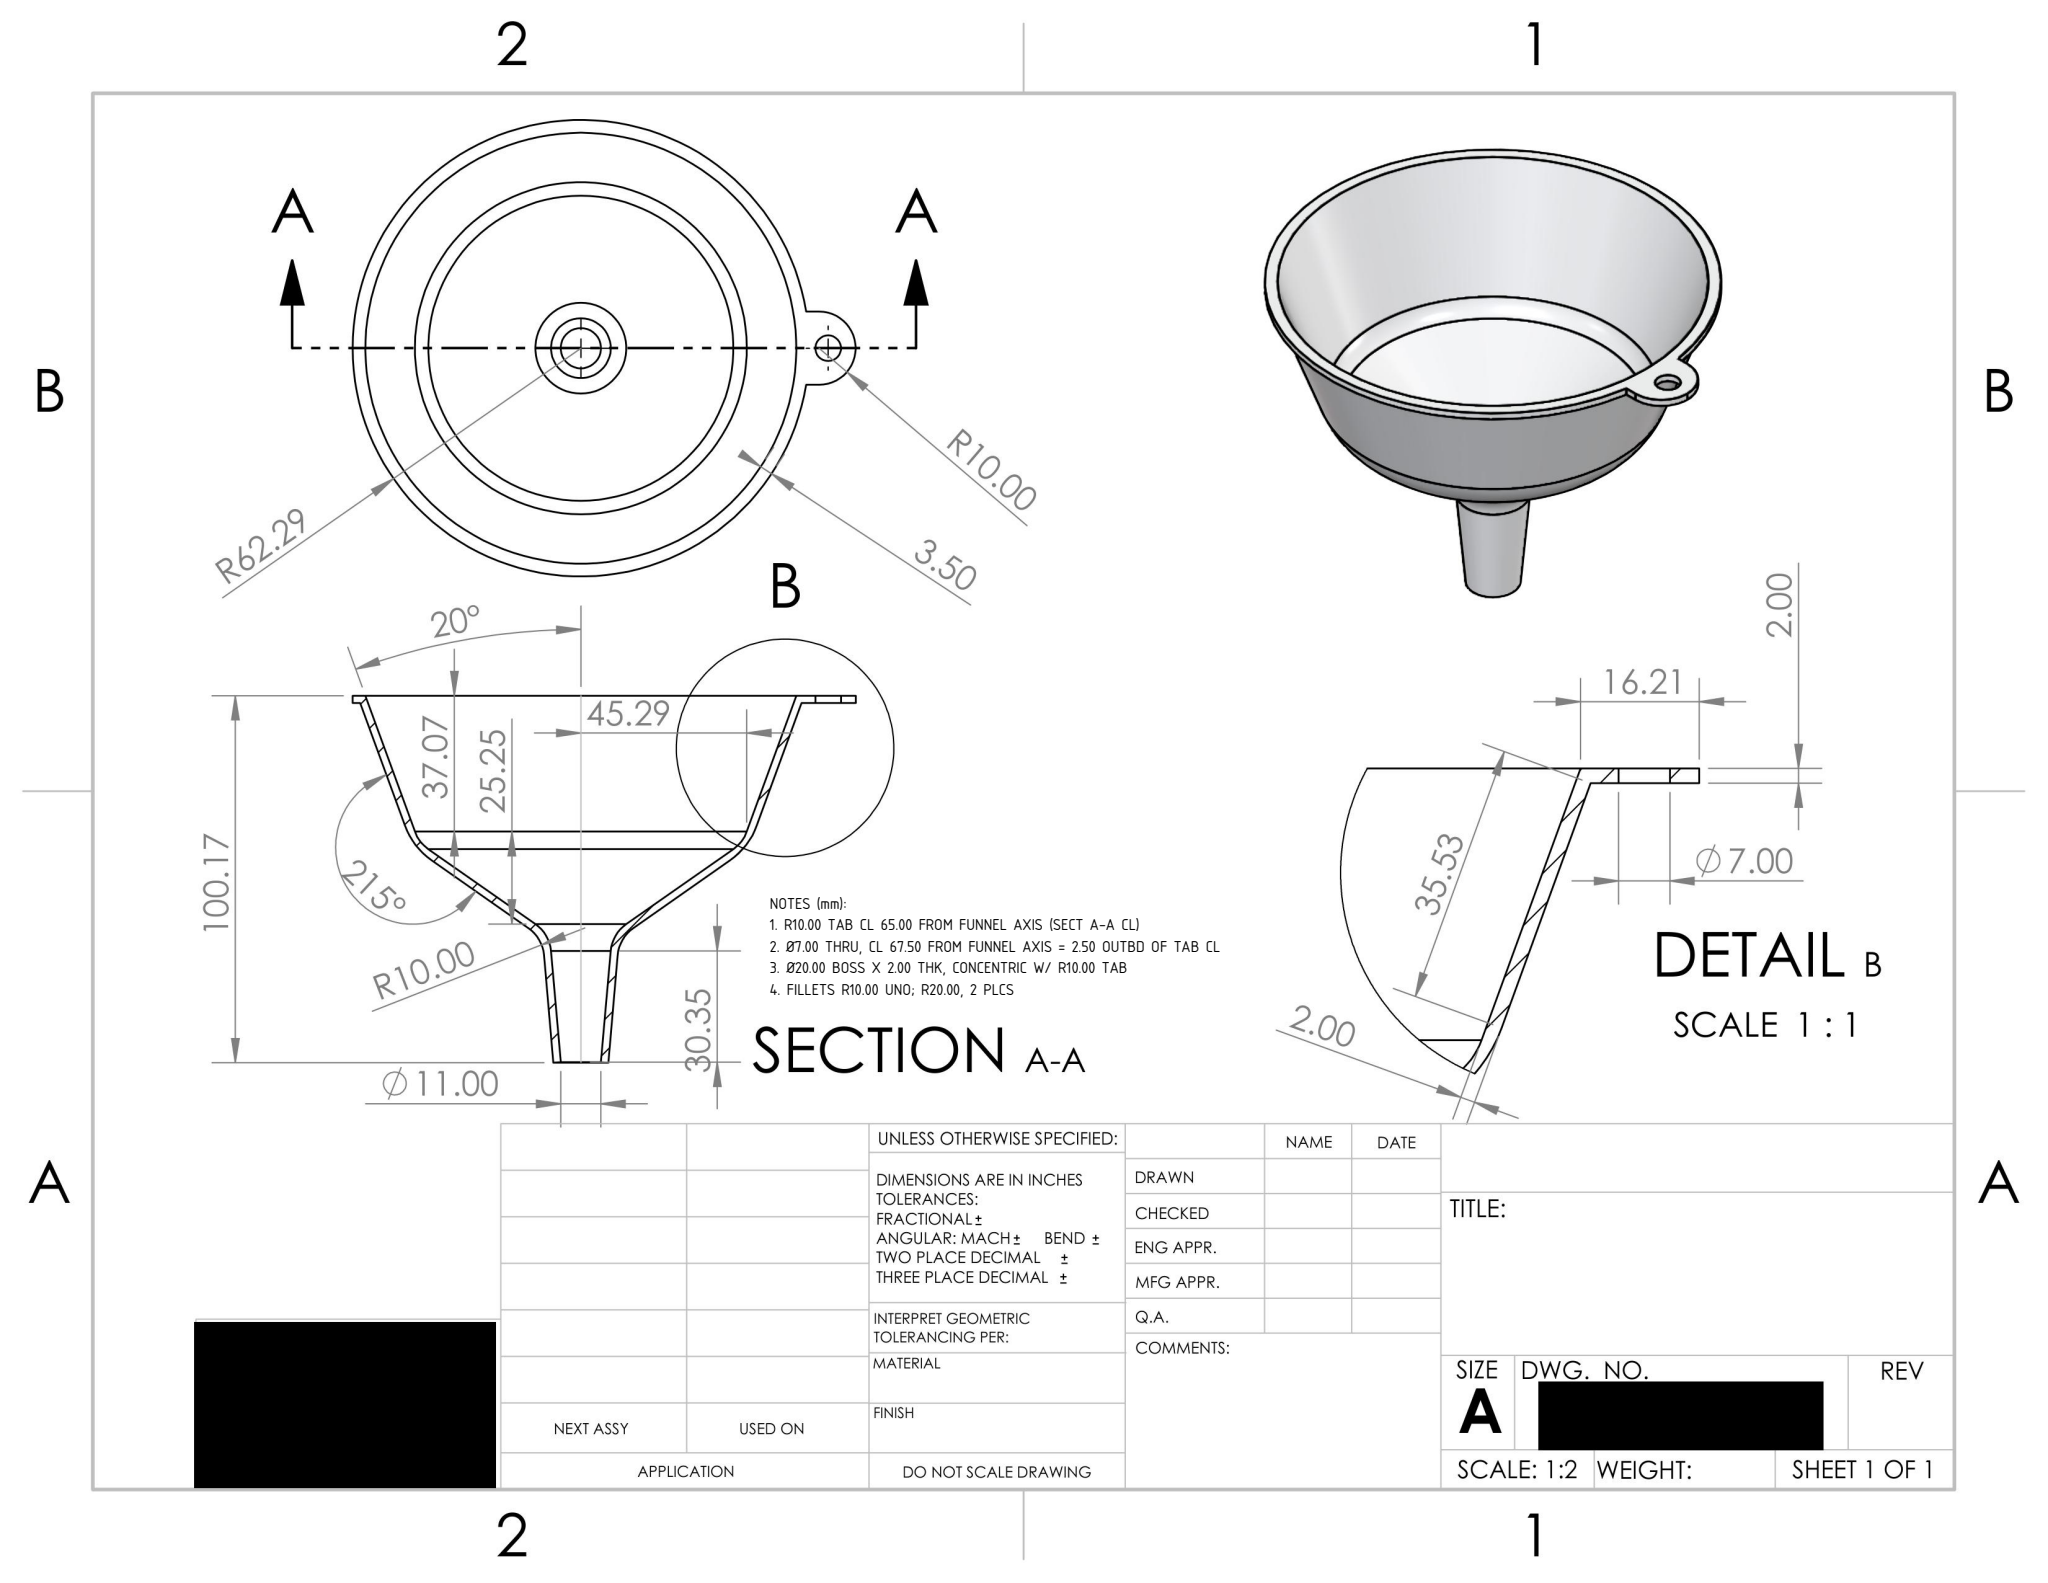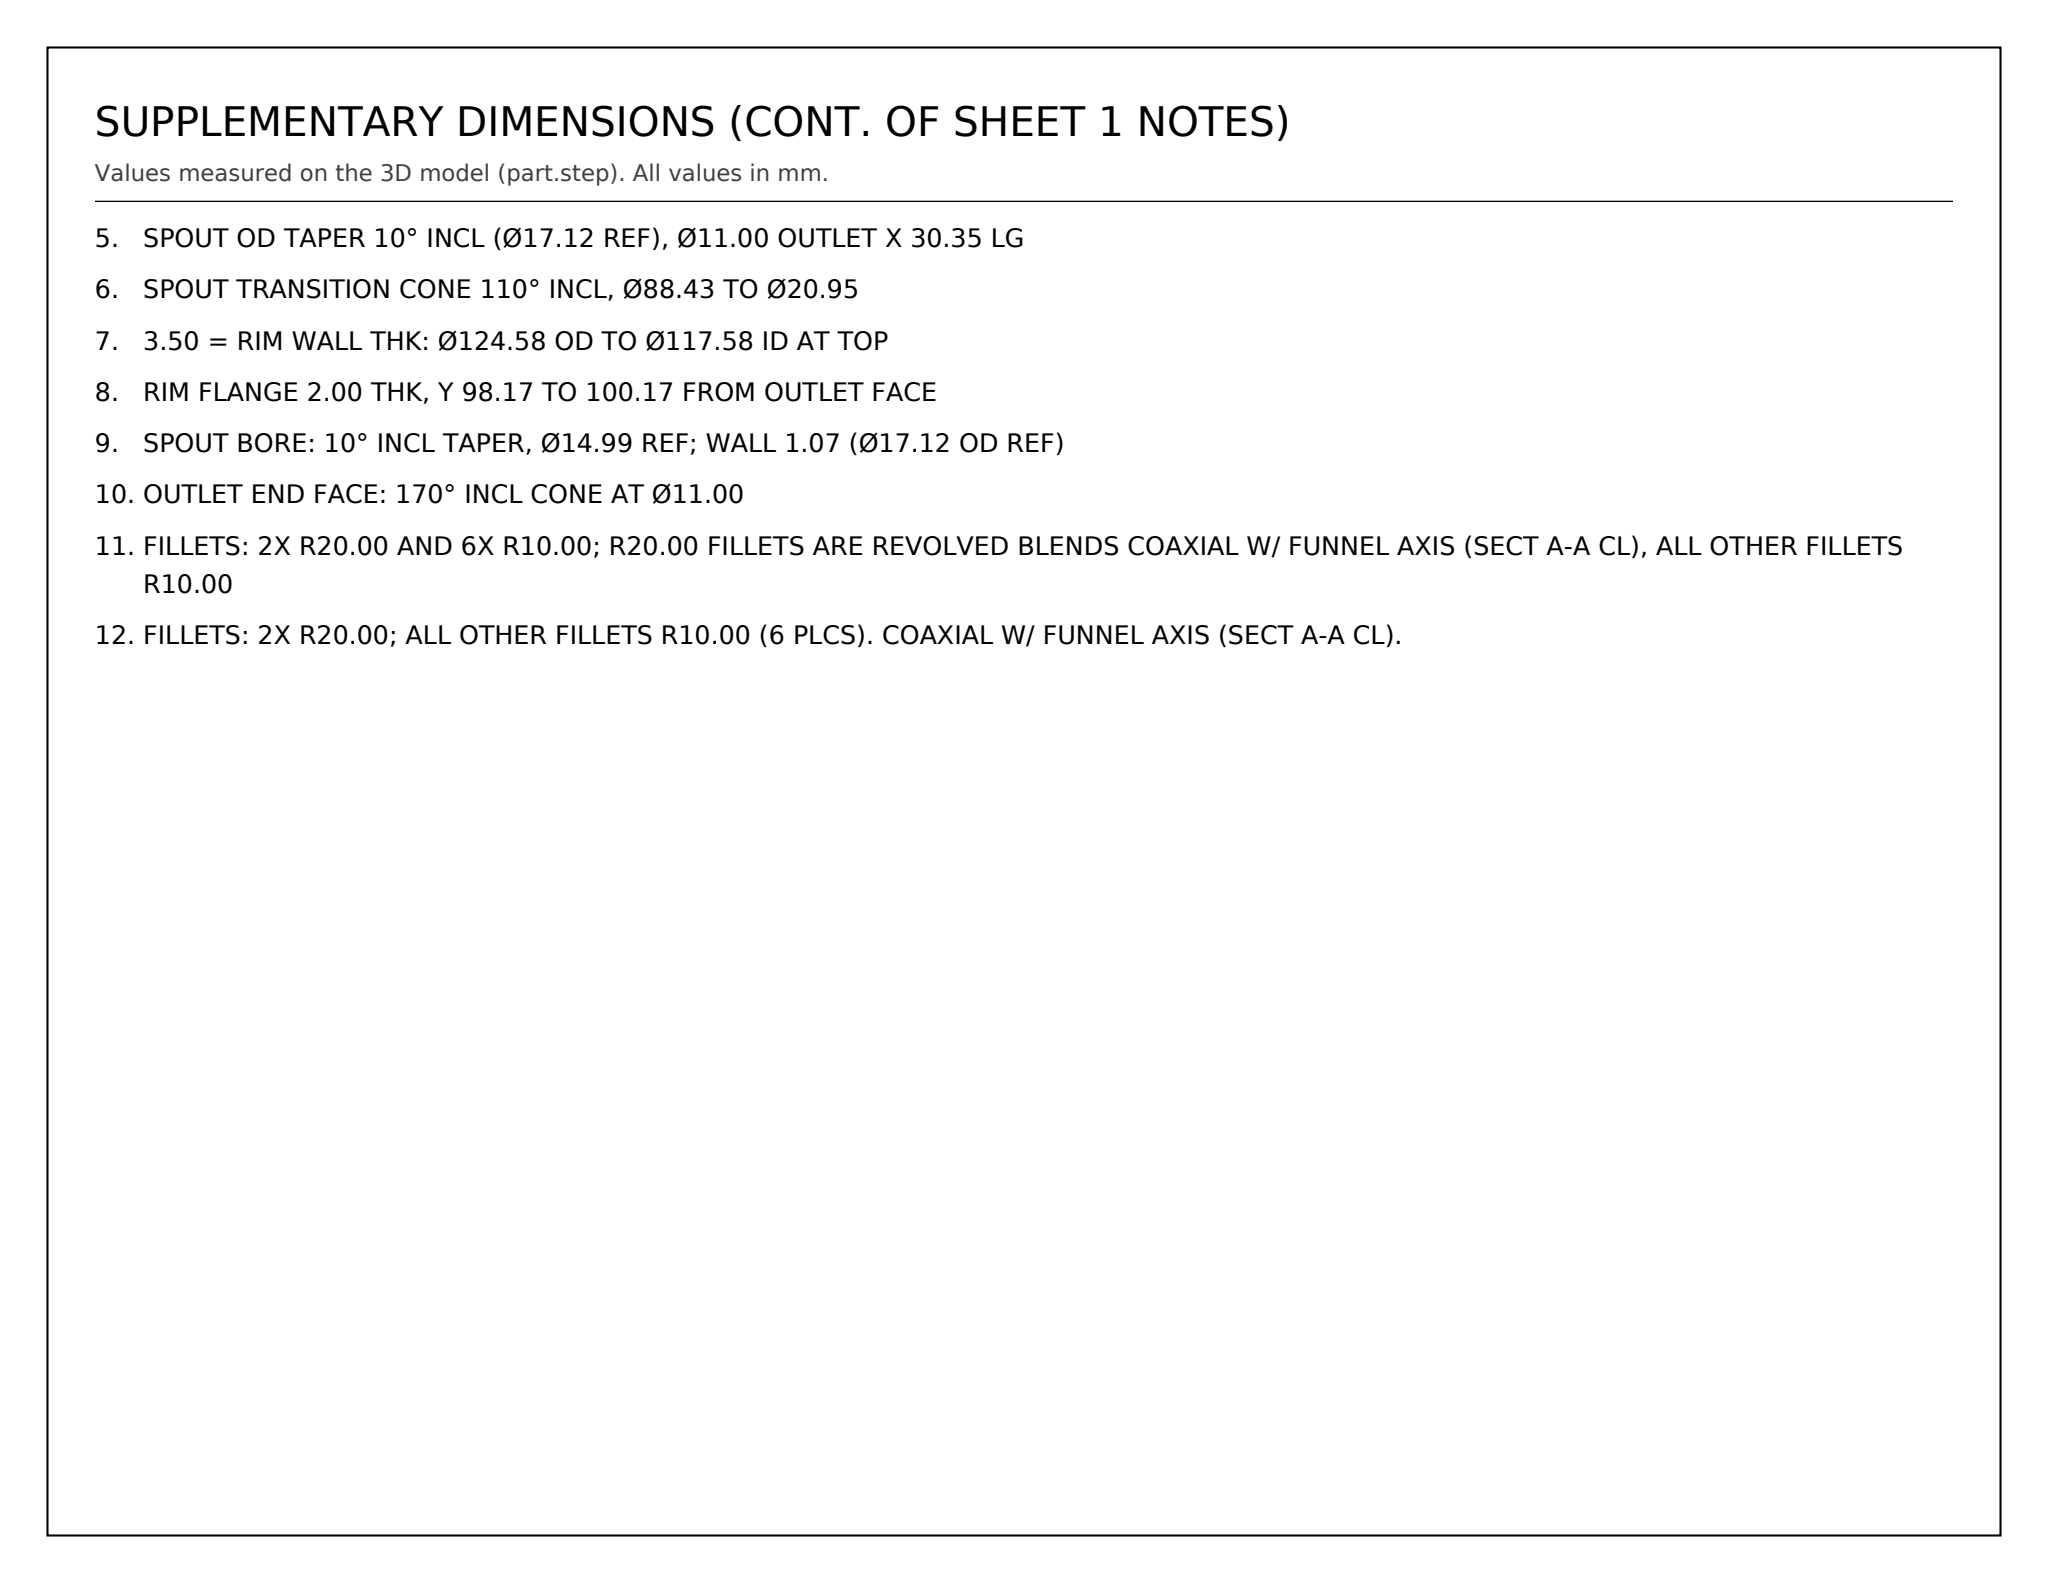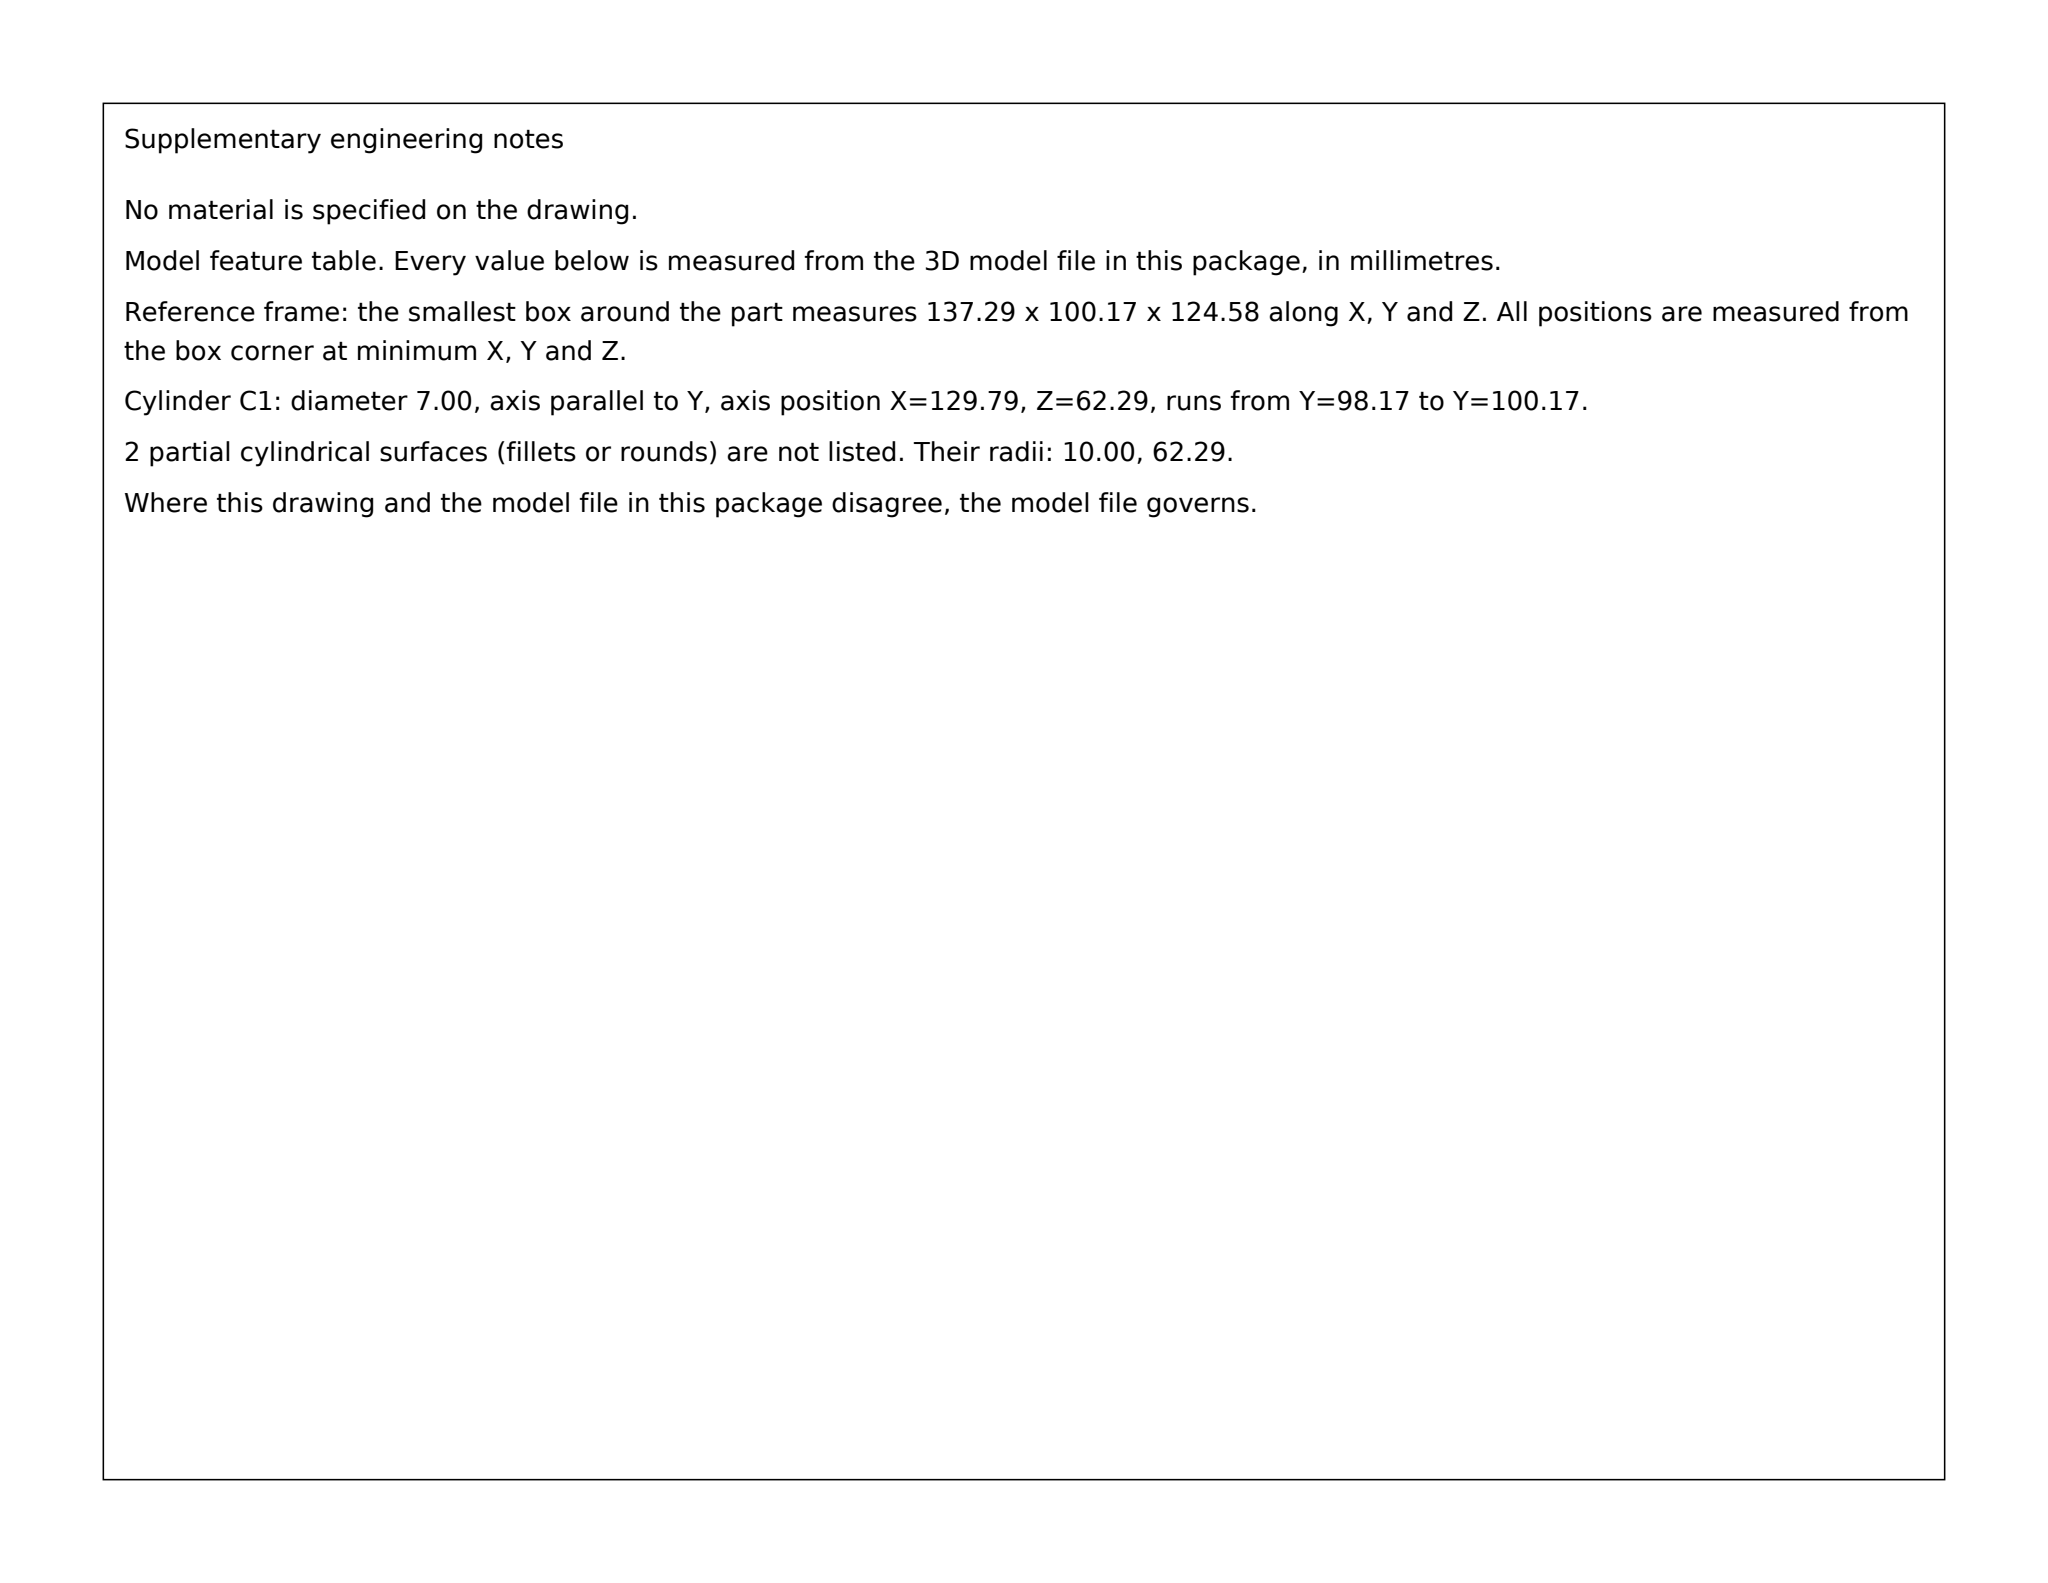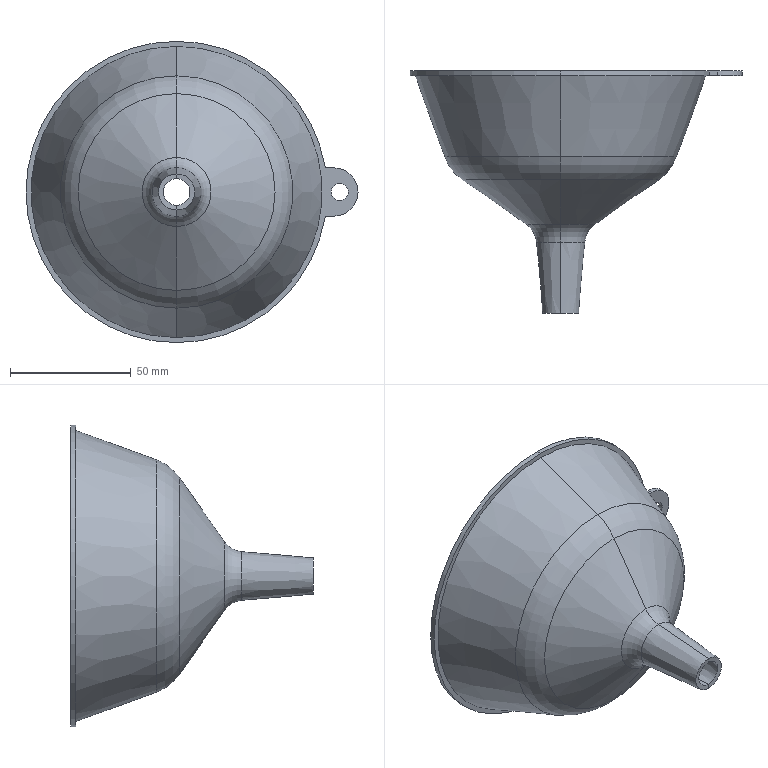Part | SolidWorks | mm | 1 solid | 33 faces | box 137.29 x 100.17 x 124.58 mm | volume 47769 mm3 | cone 14 | torus 8 | cylinder 7 | plane 4 | commonest cylinder face diameters 124.575 x3 7 x2 20 x2
Drawing notes:
R10.00 TAB CL 65.00 FROM FUNNEL AXIS (SECT A-A CL) | from the solid: Ø20 boss/tab cyl axis at x=127.29, z=62.29; funnel axis x=62.29 -> 65.00
Ø7.00 THRU, CL 67.50 FROM FUNNEL AXIS = 2.50 OUTBD OF TAB CL | from the solid: Ø7 cyl axis at x=129.79, z=62.29; 129.79-62.29=67.50; 129.79-127.29=2.50
Ø20.00 BOSS X 2.00 THK, CONCENTRIC W/ R10.00 TAB | from the solid: cylinder [20.0,'y',[127.29,null,62.29],2.0]
FILLETS R10.00 UNO; R20.00, 2 PLCS | from the solid: fillet_radii [[10.0,6],[20.0,2]]
SPOUT OD TAPER 10° INCL (Ø17.12 REF), Ø11.00 OUTLET X 30.35 LG | from the solid: cones [10.0,17.124] outer, [10.0,14.985] inner; Ø11.00 outlet
SPOUT TRANSITION CONE 110° INCL, Ø88.43 TO Ø20.95 | from the solid: cones [110.0,88.432] and [110.0,20.946]
3.50 = RIM WALL THK: Ø124.58 OD TO Ø117.58 ID AT TOP | from the solid: cylinder dia 124.575; 40° cone ref dia 117.575; (124.575-117.575)/2=3.50
RIM FLANGE 2.00 THK, Y 98.17 TO 100.17 FROM OUTLET FACE | from the solid: axis_planes ['y',98.17] and ['y',100.17]; bbox_y=100.174
SPOUT BORE: 10° INCL TAPER, Ø14.99 REF; WALL 1.07 (Ø17.12 OD REF) | from the solid: cones [10.0, 14.985] inner spout taper and [10.0, 17.124] outer spout taper; (17.124-14.985)/2=1.07
OUTLET END FACE: 170° INCL CONE AT Ø11.00 | from the solid: cones [170.0, 11.0] at spout outlet, matching Ø11.00 callout in SECTION A-A
FILLETS: 2X R20.00 AND 6X R10.00; R20.00 FILLETS ARE REVOLVED BLENDS COAXIAL W/ FUNNEL AXIS (SECT A-A CL), ALL OTHER FILLETS R10.00 | from the solid: fillet_radii: [20.0, 2] and [10.0, 6]
FILLETS: 2X R20.00; ALL OTHER FILLETS R10.00 (6 PLCS). COAXIAL W/ FUNNEL AXIS (SECT A-A CL). | from the solid: fillet_radii: [[10.0,6],[20.0,2]]